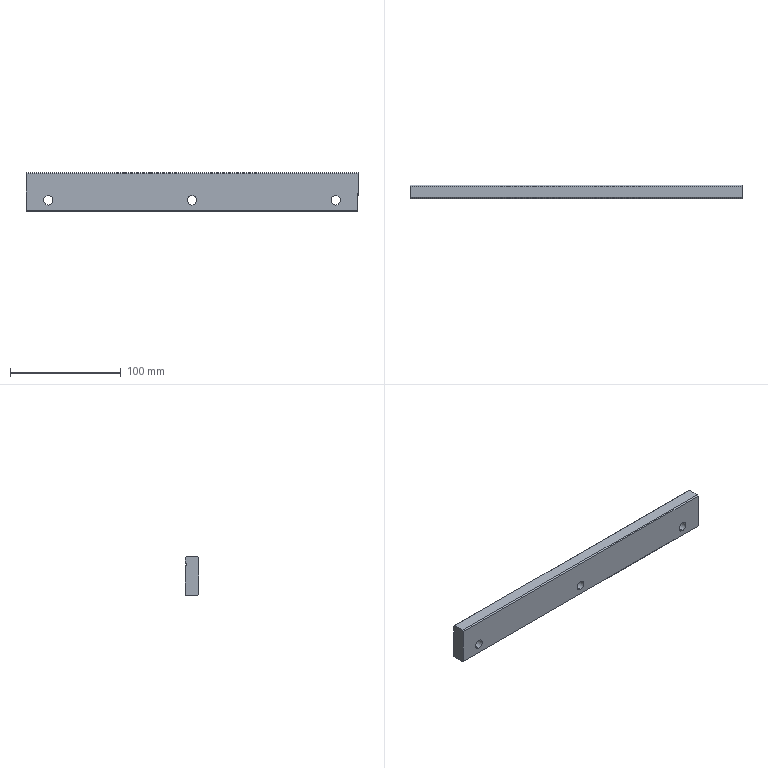Component | SolidWorks | 9LeftPressurePlate-1 | 1 solid | 19 faces | box 300 x 12 x 35 mm | volume 122907 mm3 | plane 13 | cylinder 6 | commonest cylinder face diameters 8.5 x6
build123d program:
from build123d import *

# Parameters (mm, degrees)
SKETCH1_W               = 300
SKETCH1_H               = 35
BOSS_EXTRUDE1_DEPTH     = 12
CUT_EXTRUDE1_DEPTH      = 301.749
CUT_EXTRUDE1_DEPTH_BACK = 301.749
SKETCH2_W               = 2
SKETCH2_H               = 2
CUT_EXTRUDE2_DEPTH      = 152.493
CUT_EXTRUDE2_DEPTH_BACK = 152.493
SKETCH3_R               = 4.25
CHAMFER1_SIZE           = 1


with BuildPart() as part:
    # Sketch1 → Boss-Extrude1 (new body)
    with BuildSketch(Plane(origin=(0, 0, 0), x_dir=(1, 0, 0), z_dir=(0, 1, 0))):
        Rectangle(SKETCH1_W, SKETCH1_H)
    extrude(amount=BOSS_EXTRUDE1_DEPTH)

    # Sketch2 → Cut-Extrude1 (cut, two sides: drawn at the far end of the back side and taken through both)
    with BuildSketch(Plane.ZY.offset(150).offset(-CUT_EXTRUDE1_DEPTH_BACK)):
        with Locations((10.5, 12)):
            Rectangle(SKETCH2_W, SKETCH2_H)
    extrude(amount=CUT_EXTRUDE1_DEPTH + CUT_EXTRUDE1_DEPTH_BACK, mode=Mode.SUBTRACT)

    # Sketch3 → Cut-Extrude2 (cut, two sides: drawn at the far end of the back side and taken through both)
    with BuildSketch(Plane(origin=(0, 12, 0), x_dir=(1, 0, 0), z_dir=(0, 1, 0)).offset(-CUT_EXTRUDE2_DEPTH_BACK)):
        with Locations(Location((-130, 7.5, 0), (0, 0, 270))):
            Circle(SKETCH3_R)
        with Locations(Location((0, 7.5, 0), (0, 0, 270))):
            Circle(SKETCH3_R)
        with Locations(Location((130, 7.5, 0), (0, 0, 270))):
            Circle(SKETCH3_R)
    extrude(amount=CUT_EXTRUDE2_DEPTH + CUT_EXTRUDE2_DEPTH_BACK, mode=Mode.SUBTRACT)

    # Chamfer1
    chamfer1_edges = [part.edges().sort_by_distance(p)[0] for p in [
        (0, 12, 17.5),
        (0, 0, 17.5),
        (0, 0, -17.5),
    ]]
    chamfer(chamfer1_edges, length=CHAMFER1_SIZE)


solid = part.part

# Placed as in the assembly
solid = solid.moved(Location((-4.717, 155, -32.5), (0, 0, 0)))
STEP:
#1=COLOUR_RGB('',0.7922,0.8196,0.9333);
#2=FILL_AREA_STYLE_COLOUR('',#1);
#3=FILL_AREA_STYLE('',(#2));
#4=SURFACE_STYLE_FILL_AREA(#3);
#5=SURFACE_SIDE_STYLE('',(#4));
#6=SURFACE_STYLE_USAGE(.BOTH.,#5);
#7=PRESENTATION_STYLE_ASSIGNMENT((#6));
#8=CARTESIAN_POINT('',(-5.304,6.102,-1.742));
#9=VERTEX_POINT('',#8);
#10=CARTESIAN_POINT('',(-5.304,6.102,-1.407));
#11=VERTEX_POINT('',#10);
#12=CARTESIAN_POINT('',(-5.304,6.102,-1.575));
#13=DIRECTION('',(0.,1.,0.));
#14=DIRECTION('',(0.,0.,1.));
#15=AXIS2_PLACEMENT_3D('',#12,#13,#14);
#16=CIRCLE('',#15,0.1673);
#17=EDGE_CURVE('',#9,#11,#16,.T.);
#18=ORIENTED_EDGE('',*,*,#17,.F.);
#19=CARTESIAN_POINT('',(-5.304,6.575,-1.742));
#20=VERTEX_POINT('',#19);
#21=CARTESIAN_POINT('',(-5.304,6.102,-1.742));
#22=DIRECTION('',(0.,1.,0.));
#23=VECTOR('',#22,39.37);
#24=LINE('',#21,#23);
#25=EDGE_CURVE('',#9,#20,#24,.T.);
#26=ORIENTED_EDGE('',*,*,#25,.T.);
#27=CARTESIAN_POINT('',(-5.304,6.575,-1.407));
#28=VERTEX_POINT('',#27);
#29=CARTESIAN_POINT('',(-5.304,6.575,-1.575));
#30=DIRECTION('',(0.,1.,0.));
#31=DIRECTION('',(0.,0.,1.));
#32=AXIS2_PLACEMENT_3D('',#29,#30,#31);
#33=CIRCLE('',#32,0.1673);
#34=EDGE_CURVE('',#20,#28,#33,.T.);
#35=ORIENTED_EDGE('',*,*,#34,.T.);
#36=CARTESIAN_POINT('',(-5.304,6.102,-1.407));
#37=DIRECTION('',(0.,1.,0.));
#38=VECTOR('',#37,39.37);
#39=LINE('',#36,#38);
#40=EDGE_CURVE('',#11,#28,#39,.T.);
#41=ORIENTED_EDGE('',*,*,#40,.F.);
#42=EDGE_LOOP('',(#18,#26,#35,#41));
#43=FACE_OUTER_BOUND('',#42,.T.);
#44=CARTESIAN_POINT('',(-5.304,6.102,-1.575));
#45=DIRECTION('',(0.,1.,0.));
#46=DIRECTION('',(0.,0.,1.));
#47=AXIS2_PLACEMENT_3D('',#44,#45,#46);
#48=CYLINDRICAL_SURFACE('',#47,0.1673);
#49=ADVANCED_FACE('',(#43),#48,.F.);
#50=CARTESIAN_POINT('',(-0.1857,6.102,-1.742));
#51=VERTEX_POINT('',#50);
#52=CARTESIAN_POINT('',(-0.1857,6.102,-1.407));
#53=VERTEX_POINT('',#52);
#54=CARTESIAN_POINT('',(-0.1857,6.102,-1.575));
#55=DIRECTION('',(0.,1.,0.));
#56=DIRECTION('',(0.,0.,1.));
#57=AXIS2_PLACEMENT_3D('',#54,#55,#56);
#58=CIRCLE('',#57,0.1673);
#59=EDGE_CURVE('',#51,#53,#58,.T.);
#60=ORIENTED_EDGE('',*,*,#59,.F.);
#61=CARTESIAN_POINT('',(-0.1857,6.575,-1.742));
#62=VERTEX_POINT('',#61);
#63=CARTESIAN_POINT('',(-0.1857,6.102,-1.742));
#64=DIRECTION('',(0.,1.,0.));
#65=VECTOR('',#64,39.37);
#66=LINE('',#63,#65);
#67=EDGE_CURVE('',#51,#62,#66,.T.);
#68=ORIENTED_EDGE('',*,*,#67,.T.);
#69=CARTESIAN_POINT('',(-0.1857,6.575,-1.407));
#70=VERTEX_POINT('',#69);
#71=CARTESIAN_POINT('',(-0.1857,6.575,-1.575));
#72=DIRECTION('',(0.,1.,0.));
#73=DIRECTION('',(0.,0.,1.));
#74=AXIS2_PLACEMENT_3D('',#71,#72,#73);
#75=CIRCLE('',#74,0.1673);
#76=EDGE_CURVE('',#62,#70,#75,.T.);
#77=ORIENTED_EDGE('',*,*,#76,.T.);
#78=CARTESIAN_POINT('',(-0.1857,6.102,-1.407));
#79=DIRECTION('',(0.,1.,0.));
#80=VECTOR('',#79,39.37);
#81=LINE('',#78,#80);
#82=EDGE_CURVE('',#53,#70,#81,.T.);
#83=ORIENTED_EDGE('',*,*,#82,.F.);
#84=EDGE_LOOP('',(#60,#68,#77,#83));
#85=FACE_OUTER_BOUND('',#84,.T.);
#86=CARTESIAN_POINT('',(-0.1857,6.102,-1.575));
#87=DIRECTION('',(0.,1.,0.));
#88=DIRECTION('',(0.,0.,1.));
#89=AXIS2_PLACEMENT_3D('',#86,#87,#88);
#90=CYLINDRICAL_SURFACE('',#89,0.1673);
#91=ADVANCED_FACE('',(#85),#90,.F.);
#92=CARTESIAN_POINT('',(4.932,6.102,-1.742));
#93=VERTEX_POINT('',#92);
#94=CARTESIAN_POINT('',(4.932,6.102,-1.407));
#95=VERTEX_POINT('',#94);
#96=CARTESIAN_POINT('',(4.932,6.102,-1.575));
#97=DIRECTION('',(0.,1.,0.));
#98=DIRECTION('',(0.,0.,1.));
#99=AXIS2_PLACEMENT_3D('',#96,#97,#98);
#100=CIRCLE('',#99,0.1673);
#101=EDGE_CURVE('',#93,#95,#100,.T.);
#102=ORIENTED_EDGE('',*,*,#101,.F.);
#103=CARTESIAN_POINT('',(4.932,6.575,-1.742));
#104=VERTEX_POINT('',#103);
#105=CARTESIAN_POINT('',(4.932,6.102,-1.742));
#106=DIRECTION('',(0.,1.,0.));
#107=VECTOR('',#106,39.37);
#108=LINE('',#105,#107);
#109=EDGE_CURVE('',#93,#104,#108,.T.);
#110=ORIENTED_EDGE('',*,*,#109,.T.);
#111=CARTESIAN_POINT('',(4.932,6.575,-1.407));
#112=VERTEX_POINT('',#111);
#113=CARTESIAN_POINT('',(4.932,6.575,-1.575));
#114=DIRECTION('',(0.,1.,0.));
#115=DIRECTION('',(0.,0.,1.));
#116=AXIS2_PLACEMENT_3D('',#113,#114,#115);
#117=CIRCLE('',#116,0.1673);
#118=EDGE_CURVE('',#104,#112,#117,.T.);
#119=ORIENTED_EDGE('',*,*,#118,.T.);
#120=CARTESIAN_POINT('',(4.932,6.102,-1.407));
#121=DIRECTION('',(0.,1.,0.));
#122=VECTOR('',#121,39.37);
#123=LINE('',#120,#122);
#124=EDGE_CURVE('',#95,#112,#123,.T.);
#125=ORIENTED_EDGE('',*,*,#124,.F.);
#126=EDGE_LOOP('',(#102,#110,#119,#125));
#127=FACE_OUTER_BOUND('',#126,.T.);
#128=CARTESIAN_POINT('',(4.932,6.102,-1.575));
#129=DIRECTION('',(0.,1.,0.));
#130=DIRECTION('',(0.,0.,1.));
#131=AXIS2_PLACEMENT_3D('',#128,#129,#130);
#132=CYLINDRICAL_SURFACE('',#131,0.1673);
#133=ADVANCED_FACE('',(#127),#132,.F.);
#134=CARTESIAN_POINT('',(-6.091,6.575,-0.8268));
#135=VERTEX_POINT('',#134);
#136=CARTESIAN_POINT('',(-6.091,6.575,-0.6299));
#137=VERTEX_POINT('',#136);
#138=CARTESIAN_POINT('',(-6.091,6.575,-1.969));
#139=DIRECTION('',(0.,0.,1.));
#140=VECTOR('',#139,39.37);
#141=LINE('',#138,#140);
#142=EDGE_CURVE('',#135,#137,#141,.T.);
#143=ORIENTED_EDGE('',*,*,#142,.T.);
#144=CARTESIAN_POINT('',(5.72,6.575,-0.6299));
#145=VERTEX_POINT('',#144);
#146=CARTESIAN_POINT('',(5.72,6.575,-0.6299));
#147=DIRECTION('',(1.,0.,0.));
#148=VECTOR('',#147,39.37);
#149=LINE('',#146,#148);
#150=EDGE_CURVE('',#137,#145,#149,.T.);
#151=ORIENTED_EDGE('',*,*,#150,.T.);
#152=CARTESIAN_POINT('',(5.72,6.575,-0.8268));
#153=VERTEX_POINT('',#152);
#154=CARTESIAN_POINT('',(5.72,6.575,-1.969));
#155=DIRECTION('',(-0.,0.,-1.));
#156=VECTOR('',#155,39.37);
#157=LINE('',#154,#156);
#158=EDGE_CURVE('',#145,#153,#157,.T.);
#159=ORIENTED_EDGE('',*,*,#158,.T.);
#160=CARTESIAN_POINT('',(-0.1857,6.575,-0.8268));
#161=DIRECTION('',(1.,0.,-0.));
#162=VECTOR('',#161,39.37);
#163=LINE('',#160,#162);
#164=EDGE_CURVE('',#135,#153,#163,.T.);
#165=ORIENTED_EDGE('',*,*,#164,.F.);
#166=EDGE_LOOP('',(#143,#151,#159,#165));
#167=FACE_OUTER_BOUND('',#166,.T.);
#168=CARTESIAN_POINT('',(-0.1857,6.575,-1.28));
#169=DIRECTION('',(0.,1.,0.));
#170=DIRECTION('',(0.,0.,1.));
#171=AXIS2_PLACEMENT_3D('',#168,#169,#170);
#172=PLANE('',#171);
#173=ADVANCED_FACE('',(#167),#172,.T.);
#174=ORIENTED_EDGE('',*,*,#158,.F.);
#175=CARTESIAN_POINT('',(5.72,6.535,-0.5906));
#176=VERTEX_POINT('',#175);
#177=CARTESIAN_POINT('',(5.72,6.575,-0.6299));
#178=DIRECTION('',(0.,-0.7071,0.7071));
#179=VECTOR('',#178,39.37);
#180=LINE('',#177,#179);
#181=EDGE_CURVE('',#145,#176,#180,.T.);
#182=ORIENTED_EDGE('',*,*,#181,.T.);
#183=CARTESIAN_POINT('',(5.72,6.142,-0.5906));
#184=VERTEX_POINT('',#183);
#185=CARTESIAN_POINT('',(5.72,6.575,-0.5906));
#186=DIRECTION('',(0.,-1.,0.));
#187=VECTOR('',#186,39.37);
#188=LINE('',#185,#187);
#189=EDGE_CURVE('',#176,#184,#188,.T.);
#190=ORIENTED_EDGE('',*,*,#189,.T.);
#191=CARTESIAN_POINT('',(5.72,6.102,-0.6299));
#192=VERTEX_POINT('',#191);
#193=CARTESIAN_POINT('',(5.72,6.142,-0.5906));
#194=DIRECTION('',(-0.,-0.7071,-0.7071));
#195=VECTOR('',#194,39.37);
#196=LINE('',#193,#195);
#197=EDGE_CURVE('',#184,#192,#196,.T.);
#198=ORIENTED_EDGE('',*,*,#197,.T.);
#199=CARTESIAN_POINT('',(5.72,6.102,-1.929));
#200=VERTEX_POINT('',#199);
#201=CARTESIAN_POINT('',(5.72,6.102,-1.969));
#202=DIRECTION('',(-0.,0.,-1.));
#203=VECTOR('',#202,39.37);
#204=LINE('',#201,#203);
#205=EDGE_CURVE('',#192,#200,#204,.T.);
#206=ORIENTED_EDGE('',*,*,#205,.T.);
#207=CARTESIAN_POINT('',(5.72,6.142,-1.969));
#208=VERTEX_POINT('',#207);
#209=CARTESIAN_POINT('',(5.72,6.142,-1.969));
#210=DIRECTION('',(-0.,0.7071,-0.7071));
#211=VECTOR('',#210,39.37);
#212=LINE('',#209,#211);
#213=EDGE_CURVE('',#200,#208,#212,.T.);
#214=ORIENTED_EDGE('',*,*,#213,.T.);
#215=CARTESIAN_POINT('',(5.72,6.575,-1.969));
#216=VERTEX_POINT('',#215);
#217=CARTESIAN_POINT('',(5.72,6.575,-1.969));
#218=DIRECTION('',(0.,-1.,0.));
#219=VECTOR('',#218,39.37);
#220=LINE('',#217,#219);
#221=EDGE_CURVE('',#216,#208,#220,.T.);
#222=ORIENTED_EDGE('',*,*,#221,.F.);
#223=CARTESIAN_POINT('',(5.72,6.575,-0.9055));
#224=VERTEX_POINT('',#223);
#225=CARTESIAN_POINT('',(5.72,6.575,-1.969));
#226=DIRECTION('',(-0.,0.,-1.));
#227=VECTOR('',#226,39.37);
#228=LINE('',#225,#227);
#229=EDGE_CURVE('',#224,#216,#228,.T.);
#230=ORIENTED_EDGE('',*,*,#229,.F.);
#231=CARTESIAN_POINT('',(5.72,6.535,-0.9055));
#232=VERTEX_POINT('',#231);
#233=CARTESIAN_POINT('',(5.72,6.614,-0.9055));
#234=DIRECTION('',(0.,-1.,0.));
#235=VECTOR('',#234,39.37);
#236=LINE('',#233,#235);
#237=EDGE_CURVE('',#224,#232,#236,.T.);
#238=ORIENTED_EDGE('',*,*,#237,.T.);
#239=CARTESIAN_POINT('',(5.72,6.535,-0.8268));
#240=VERTEX_POINT('',#239);
#241=CARTESIAN_POINT('',(5.72,6.535,-0.9055));
#242=DIRECTION('',(0.,0.,1.));
#243=VECTOR('',#242,39.37);
#244=LINE('',#241,#243);
#245=EDGE_CURVE('',#232,#240,#244,.T.);
#246=ORIENTED_EDGE('',*,*,#245,.T.);
#247=CARTESIAN_POINT('',(5.72,6.614,-0.8268));
#248=DIRECTION('',(0.,1.,0.));
#249=VECTOR('',#248,39.37);
#250=LINE('',#247,#249);
#251=EDGE_CURVE('',#240,#153,#250,.T.);
#252=ORIENTED_EDGE('',*,*,#251,.T.);
#253=EDGE_LOOP('',(#174,#182,#190,#198,#206,#214,#222,#230,#238,#246,#252));
#254=FACE_OUTER_BOUND('',#253,.T.);
#255=CARTESIAN_POINT('',(5.72,6.575,-1.969));
#256=DIRECTION('',(-1.,0.,0.));
#257=DIRECTION('',(0.,0.,1.));
#258=AXIS2_PLACEMENT_3D('',#255,#256,#257);
#259=PLANE('',#258);
#260=ADVANCED_FACE('',(#254),#259,.F.);
#261=ORIENTED_EDGE('',*,*,#221,.T.);
#262=CARTESIAN_POINT('',(-6.091,6.142,-1.969));
#263=VERTEX_POINT('',#262);
#264=CARTESIAN_POINT('',(-6.091,6.142,-1.969));
#265=DIRECTION('',(-1.,0.,0.));
#266=VECTOR('',#265,39.37);
#267=LINE('',#264,#266);
#268=EDGE_CURVE('',#208,#263,#267,.T.);
#269=ORIENTED_EDGE('',*,*,#268,.T.);
#270=CARTESIAN_POINT('',(-6.091,6.575,-1.969));
#271=VERTEX_POINT('',#270);
#272=CARTESIAN_POINT('',(-6.091,6.575,-1.969));
#273=DIRECTION('',(0.,-1.,0.));
#274=VECTOR('',#273,39.37);
#275=LINE('',#272,#274);
#276=EDGE_CURVE('',#271,#263,#275,.T.);
#277=ORIENTED_EDGE('',*,*,#276,.F.);
#278=CARTESIAN_POINT('',(-6.091,6.575,-1.969));
#279=DIRECTION('',(-1.,0.,0.));
#280=VECTOR('',#279,39.37);
#281=LINE('',#278,#280);
#282=EDGE_CURVE('',#216,#271,#281,.T.);
#283=ORIENTED_EDGE('',*,*,#282,.F.);
#284=EDGE_LOOP('',(#261,#269,#277,#283));
#285=FACE_OUTER_BOUND('',#284,.T.);
#286=CARTESIAN_POINT('',(-6.091,6.575,-1.969));
#287=DIRECTION('',(0.,0.,1.));
#288=DIRECTION('',(1.,0.,0.));
#289=AXIS2_PLACEMENT_3D('',#286,#287,#288);
#290=PLANE('',#289);
#291=ADVANCED_FACE('',(#285),#290,.F.);
#292=CARTESIAN_POINT('',(-6.091,6.535,-0.5906));
#293=VERTEX_POINT('',#292);
#294=CARTESIAN_POINT('',(-6.091,6.142,-0.5906));
#295=VERTEX_POINT('',#294);
#296=CARTESIAN_POINT('',(-6.091,6.575,-0.5906));
#297=DIRECTION('',(0.,-1.,0.));
#298=VECTOR('',#297,39.37);
#299=LINE('',#296,#298);
#300=EDGE_CURVE('',#293,#295,#299,.T.);
#301=ORIENTED_EDGE('',*,*,#300,.F.);
#302=CARTESIAN_POINT('',(-6.091,6.575,-0.6299));
#303=DIRECTION('',(-0.,0.7071,-0.7071));
#304=VECTOR('',#303,39.37);
#305=LINE('',#302,#304);
#306=EDGE_CURVE('',#293,#137,#305,.T.);
#307=ORIENTED_EDGE('',*,*,#306,.T.);
#308=ORIENTED_EDGE('',*,*,#142,.F.);
#309=CARTESIAN_POINT('',(-6.091,6.535,-0.8268));
#310=VERTEX_POINT('',#309);
#311=CARTESIAN_POINT('',(-6.091,6.575,-0.8268));
#312=DIRECTION('',(0.,-1.,0.));
#313=VECTOR('',#312,39.37);
#314=LINE('',#311,#313);
#315=EDGE_CURVE('',#135,#310,#314,.T.);
#316=ORIENTED_EDGE('',*,*,#315,.T.);
#317=CARTESIAN_POINT('',(-6.091,6.535,-0.9055));
#318=VERTEX_POINT('',#317);
#319=CARTESIAN_POINT('',(-6.091,6.535,-1.969));
#320=DIRECTION('',(-0.,0.,-1.));
#321=VECTOR('',#320,39.37);
#322=LINE('',#319,#321);
#323=EDGE_CURVE('',#310,#318,#322,.T.);
#324=ORIENTED_EDGE('',*,*,#323,.T.);
#325=CARTESIAN_POINT('',(-6.091,6.575,-0.9055));
#326=VERTEX_POINT('',#325);
#327=CARTESIAN_POINT('',(-6.091,6.575,-0.9055));
#328=DIRECTION('',(0.,1.,0.));
#329=VECTOR('',#328,39.37);
#330=LINE('',#327,#329);
#331=EDGE_CURVE('',#318,#326,#330,.T.);
#332=ORIENTED_EDGE('',*,*,#331,.T.);
#333=CARTESIAN_POINT('',(-6.091,6.575,-1.969));
#334=DIRECTION('',(0.,0.,1.));
#335=VECTOR('',#334,39.37);
#336=LINE('',#333,#335);
#337=EDGE_CURVE('',#271,#326,#336,.T.);
#338=ORIENTED_EDGE('',*,*,#337,.F.);
#339=ORIENTED_EDGE('',*,*,#276,.T.);
#340=CARTESIAN_POINT('',(-6.091,6.102,-1.929));
#341=VERTEX_POINT('',#340);
#342=CARTESIAN_POINT('',(-6.091,6.142,-1.969));
#343=DIRECTION('',(0.,-0.7071,0.7071));
#344=VECTOR('',#343,39.37);
#345=LINE('',#342,#344);
#346=EDGE_CURVE('',#263,#341,#345,.T.);
#347=ORIENTED_EDGE('',*,*,#346,.T.);
#348=CARTESIAN_POINT('',(-6.091,6.102,-0.6299));
#349=VERTEX_POINT('',#348);
#350=CARTESIAN_POINT('',(-6.091,6.102,-1.969));
#351=DIRECTION('',(0.,0.,1.));
#352=VECTOR('',#351,39.37);
#353=LINE('',#350,#352);
#354=EDGE_CURVE('',#341,#349,#353,.T.);
#355=ORIENTED_EDGE('',*,*,#354,.T.);
#356=CARTESIAN_POINT('',(-6.091,6.142,-0.5906));
#357=DIRECTION('',(0.,0.7071,0.7071));
#358=VECTOR('',#357,39.37);
#359=LINE('',#356,#358);
#360=EDGE_CURVE('',#349,#295,#359,.T.);
#361=ORIENTED_EDGE('',*,*,#360,.T.);
#362=EDGE_LOOP('',(#301,#307,#308,#316,#324,#332,#338,#339,#347,#355,#361));
#363=FACE_OUTER_BOUND('',#362,.T.);
#364=CARTESIAN_POINT('',(-6.091,6.575,-1.969));
#365=DIRECTION('',(1.,0.,-0.));
#366=DIRECTION('',(-0.,0.,-1.));
#367=AXIS2_PLACEMENT_3D('',#364,#365,#366);
#368=PLANE('',#367);
#369=ADVANCED_FACE('',(#363),#368,.F.);
#370=ORIENTED_EDGE('',*,*,#189,.F.);
#371=CARTESIAN_POINT('',(-6.091,6.535,-0.5906));
#372=DIRECTION('',(-1.,0.,0.));
#373=VECTOR('',#372,39.37);
#374=LINE('',#371,#373);
#375=EDGE_CURVE('',#176,#293,#374,.T.);
#376=ORIENTED_EDGE('',*,*,#375,.T.);
#377=ORIENTED_EDGE('',*,*,#300,.T.);
#378=CARTESIAN_POINT('',(-6.091,6.142,-0.5906));
#379=DIRECTION('',(1.,0.,0.));
#380=VECTOR('',#379,39.37);
#381=LINE('',#378,#380);
#382=EDGE_CURVE('',#295,#184,#381,.T.);
#383=ORIENTED_EDGE('',*,*,#382,.T.);
#384=EDGE_LOOP('',(#370,#376,#377,#383));
#385=FACE_OUTER_BOUND('',#384,.T.);
#386=CARTESIAN_POINT('',(-6.091,6.575,-0.5906));
#387=DIRECTION('',(0.,0.,-1.));
#388=DIRECTION('',(-1.,0.,0.));
#389=AXIS2_PLACEMENT_3D('',#386,#387,#388);
#390=PLANE('',#389);
#391=ADVANCED_FACE('',(#385),#390,.F.);
#392=CARTESIAN_POINT('',(-5.304,6.575,-1.575));
#393=DIRECTION('',(0.,1.,0.));
#394=DIRECTION('',(0.,0.,1.));
#395=AXIS2_PLACEMENT_3D('',#392,#393,#394);
#396=CIRCLE('',#395,0.1673);
#397=EDGE_CURVE('',#28,#20,#396,.T.);
#398=ORIENTED_EDGE('',*,*,#397,.F.);
#399=ORIENTED_EDGE('',*,*,#34,.F.);
#400=EDGE_LOOP('',(#398,#399));
#401=FACE_BOUND('',#400,.T.);
#402=CARTESIAN_POINT('',(-0.1857,6.575,-1.575));
#403=DIRECTION('',(0.,1.,0.));
#404=DIRECTION('',(0.,0.,1.));
#405=AXIS2_PLACEMENT_3D('',#402,#403,#404);
#406=CIRCLE('',#405,0.1673);
#407=EDGE_CURVE('',#70,#62,#406,.T.);
#408=ORIENTED_EDGE('',*,*,#407,.F.);
#409=ORIENTED_EDGE('',*,*,#76,.F.);
#410=EDGE_LOOP('',(#408,#409));
#411=FACE_BOUND('',#410,.T.);
#412=CARTESIAN_POINT('',(4.932,6.575,-1.575));
#413=DIRECTION('',(0.,1.,0.));
#414=DIRECTION('',(0.,0.,1.));
#415=AXIS2_PLACEMENT_3D('',#412,#413,#414);
#416=CIRCLE('',#415,0.1673);
#417=EDGE_CURVE('',#112,#104,#416,.T.);
#418=ORIENTED_EDGE('',*,*,#417,.F.);
#419=ORIENTED_EDGE('',*,*,#118,.F.);
#420=EDGE_LOOP('',(#418,#419));
#421=FACE_BOUND('',#420,.T.);
#422=CARTESIAN_POINT('',(-0.1857,6.575,-0.9055));
#423=DIRECTION('',(-1.,0.,0.));
#424=VECTOR('',#423,39.37);
#425=LINE('',#422,#424);
#426=EDGE_CURVE('',#224,#326,#425,.T.);
#427=ORIENTED_EDGE('',*,*,#426,.F.);
#428=ORIENTED_EDGE('',*,*,#229,.T.);
#429=ORIENTED_EDGE('',*,*,#282,.T.);
#430=ORIENTED_EDGE('',*,*,#337,.T.);
#431=EDGE_LOOP('',(#427,#428,#429,#430));
#432=FACE_OUTER_BOUND('',#431,.T.);
#433=CARTESIAN_POINT('',(-0.1857,6.575,-1.28));
#434=DIRECTION('',(0.,1.,0.));
#435=DIRECTION('',(0.,0.,1.));
#436=AXIS2_PLACEMENT_3D('',#433,#434,#435);
#437=PLANE('',#436);
#438=ADVANCED_FACE('',(#401,#411,#421,#432),#437,.T.);
#439=CARTESIAN_POINT('',(-5.304,6.102,-1.575));
#440=DIRECTION('',(0.,1.,0.));
#441=DIRECTION('',(0.,0.,1.));
#442=AXIS2_PLACEMENT_3D('',#439,#440,#441);
#443=CIRCLE('',#442,0.1673);
#444=EDGE_CURVE('',#11,#9,#443,.T.);
#445=ORIENTED_EDGE('',*,*,#444,.T.);
#446=ORIENTED_EDGE('',*,*,#17,.T.);
#447=EDGE_LOOP('',(#445,#446));
#448=FACE_BOUND('',#447,.T.);
#449=CARTESIAN_POINT('',(-0.1857,6.102,-1.575));
#450=DIRECTION('',(0.,1.,0.));
#451=DIRECTION('',(0.,0.,1.));
#452=AXIS2_PLACEMENT_3D('',#449,#450,#451);
#453=CIRCLE('',#452,0.1673);
#454=EDGE_CURVE('',#53,#51,#453,.T.);
#455=ORIENTED_EDGE('',*,*,#454,.T.);
#456=ORIENTED_EDGE('',*,*,#59,.T.);
#457=EDGE_LOOP('',(#455,#456));
#458=FACE_BOUND('',#457,.T.);
#459=CARTESIAN_POINT('',(4.932,6.102,-1.575));
#460=DIRECTION('',(0.,1.,0.));
#461=DIRECTION('',(0.,0.,1.));
#462=AXIS2_PLACEMENT_3D('',#459,#460,#461);
#463=CIRCLE('',#462,0.1673);
#464=EDGE_CURVE('',#95,#93,#463,.T.);
#465=ORIENTED_EDGE('',*,*,#464,.T.);
#466=ORIENTED_EDGE('',*,*,#101,.T.);
#467=EDGE_LOOP('',(#465,#466));
#468=FACE_BOUND('',#467,.T.);
#469=ORIENTED_EDGE('',*,*,#205,.F.);
#470=CARTESIAN_POINT('',(-0.1857,6.102,-0.6299));
#471=DIRECTION('',(-1.,0.,0.));
#472=VECTOR('',#471,39.37);
#473=LINE('',#470,#472);
#474=EDGE_CURVE('',#192,#349,#473,.T.);
#475=ORIENTED_EDGE('',*,*,#474,.T.);
#476=ORIENTED_EDGE('',*,*,#354,.F.);
#477=CARTESIAN_POINT('',(-0.1857,6.102,-1.929));
#478=DIRECTION('',(1.,0.,0.));
#479=VECTOR('',#478,39.37);
#480=LINE('',#477,#479);
#481=EDGE_CURVE('',#341,#200,#480,.T.);
#482=ORIENTED_EDGE('',*,*,#481,.T.);
#483=EDGE_LOOP('',(#469,#475,#476,#482));
#484=FACE_OUTER_BOUND('',#483,.T.);
#485=CARTESIAN_POINT('',(-0.1857,6.102,-1.28));
#486=DIRECTION('',(0.,1.,0.));
#487=DIRECTION('',(0.,0.,1.));
#488=AXIS2_PLACEMENT_3D('',#485,#486,#487);
#489=PLANE('',#488);
#490=ADVANCED_FACE('',(#448,#458,#468,#484),#489,.F.);
#491=CARTESIAN_POINT('',(5.72,6.535,-0.8268));
#492=DIRECTION('',(-1.,0.,0.));
#493=VECTOR('',#492,39.37);
#494=LINE('',#491,#493);
#495=EDGE_CURVE('',#240,#310,#494,.T.);
#496=ORIENTED_EDGE('',*,*,#495,.F.);
#497=ORIENTED_EDGE('',*,*,#245,.F.);
#498=CARTESIAN_POINT('',(5.72,6.535,-0.9055));
#499=DIRECTION('',(-1.,0.,0.));
#500=VECTOR('',#499,39.37);
#501=LINE('',#498,#500);
#502=EDGE_CURVE('',#232,#318,#501,.T.);
#503=ORIENTED_EDGE('',*,*,#502,.T.);
#504=ORIENTED_EDGE('',*,*,#323,.F.);
#505=EDGE_LOOP('',(#496,#497,#503,#504));
#506=FACE_OUTER_BOUND('',#505,.T.);
#507=CARTESIAN_POINT('',(5.72,6.535,-0.9055));
#508=DIRECTION('',(0.,-1.,0.));
#509=DIRECTION('',(0.,0.,-1.));
#510=AXIS2_PLACEMENT_3D('',#507,#508,#509);
#511=PLANE('',#510);
#512=ADVANCED_FACE('',(#506),#511,.F.);
#513=ORIENTED_EDGE('',*,*,#164,.T.);
#514=ORIENTED_EDGE('',*,*,#251,.F.);
#515=ORIENTED_EDGE('',*,*,#495,.T.);
#516=ORIENTED_EDGE('',*,*,#315,.F.);
#517=EDGE_LOOP('',(#513,#514,#515,#516));
#518=FACE_OUTER_BOUND('',#517,.T.);
#519=CARTESIAN_POINT('',(5.72,6.614,-0.8268));
#520=DIRECTION('',(0.,0.,1.));
#521=DIRECTION('',(1.,0.,-0.));
#522=AXIS2_PLACEMENT_3D('',#519,#520,#521);
#523=PLANE('',#522);
#524=ADVANCED_FACE('',(#518),#523,.F.);
#525=ORIENTED_EDGE('',*,*,#502,.F.);
#526=ORIENTED_EDGE('',*,*,#237,.F.);
#527=ORIENTED_EDGE('',*,*,#426,.T.);
#528=ORIENTED_EDGE('',*,*,#331,.F.);
#529=EDGE_LOOP('',(#525,#526,#527,#528));
#530=FACE_OUTER_BOUND('',#529,.T.);
#531=CARTESIAN_POINT('',(5.72,6.614,-0.9055));
#532=DIRECTION('',(-0.,0.,-1.));
#533=DIRECTION('',(-1.,0.,0.));
#534=AXIS2_PLACEMENT_3D('',#531,#532,#533);
#535=PLANE('',#534);
#536=ADVANCED_FACE('',(#530),#535,.F.);
#537=ORIENTED_EDGE('',*,*,#109,.F.);
#538=ORIENTED_EDGE('',*,*,#464,.F.);
#539=ORIENTED_EDGE('',*,*,#124,.T.);
#540=ORIENTED_EDGE('',*,*,#417,.T.);
#541=EDGE_LOOP('',(#537,#538,#539,#540));
#542=FACE_OUTER_BOUND('',#541,.T.);
#543=CARTESIAN_POINT('',(4.932,6.102,-1.575));
#544=DIRECTION('',(0.,1.,0.));
#545=DIRECTION('',(0.,0.,1.));
#546=AXIS2_PLACEMENT_3D('',#543,#544,#545);
#547=CYLINDRICAL_SURFACE('',#546,0.1673);
#548=ADVANCED_FACE('',(#542),#547,.F.);
#549=ORIENTED_EDGE('',*,*,#67,.F.);
#550=ORIENTED_EDGE('',*,*,#454,.F.);
#551=ORIENTED_EDGE('',*,*,#82,.T.);
#552=ORIENTED_EDGE('',*,*,#407,.T.);
#553=EDGE_LOOP('',(#549,#550,#551,#552));
#554=FACE_OUTER_BOUND('',#553,.T.);
#555=CARTESIAN_POINT('',(-0.1857,6.102,-1.575));
#556=DIRECTION('',(0.,1.,0.));
#557=DIRECTION('',(0.,0.,1.));
#558=AXIS2_PLACEMENT_3D('',#555,#556,#557);
#559=CYLINDRICAL_SURFACE('',#558,0.1673);
#560=ADVANCED_FACE('',(#554),#559,.F.);
#561=ORIENTED_EDGE('',*,*,#25,.F.);
#562=ORIENTED_EDGE('',*,*,#444,.F.);
#563=ORIENTED_EDGE('',*,*,#40,.T.);
#564=ORIENTED_EDGE('',*,*,#397,.T.);
#565=EDGE_LOOP('',(#561,#562,#563,#564));
#566=FACE_OUTER_BOUND('',#565,.T.);
#567=CARTESIAN_POINT('',(-5.304,6.102,-1.575));
#568=DIRECTION('',(0.,1.,0.));
#569=DIRECTION('',(0.,0.,1.));
#570=AXIS2_PLACEMENT_3D('',#567,#568,#569);
#571=CYLINDRICAL_SURFACE('',#570,0.1673);
#572=ADVANCED_FACE('',(#566),#571,.F.);
#573=ORIENTED_EDGE('',*,*,#306,.F.);
#574=ORIENTED_EDGE('',*,*,#375,.F.);
#575=ORIENTED_EDGE('',*,*,#181,.F.);
#576=ORIENTED_EDGE('',*,*,#150,.F.);
#577=EDGE_LOOP('',(#573,#574,#575,#576));
#578=FACE_OUTER_BOUND('',#577,.T.);
#579=CARTESIAN_POINT('',(-0.1857,6.575,-0.6299));
#580=DIRECTION('',(0.,0.7071,0.7071));
#581=DIRECTION('',(-1.,0.,0.));
#582=AXIS2_PLACEMENT_3D('',#579,#580,#581);
#583=PLANE('',#582);
#584=ADVANCED_FACE('',(#578),#583,.T.);
#585=ORIENTED_EDGE('',*,*,#360,.F.);
#586=ORIENTED_EDGE('',*,*,#474,.F.);
#587=ORIENTED_EDGE('',*,*,#197,.F.);
#588=ORIENTED_EDGE('',*,*,#382,.F.);
#589=EDGE_LOOP('',(#585,#586,#587,#588));
#590=FACE_OUTER_BOUND('',#589,.T.);
#591=CARTESIAN_POINT('',(-6.091,6.142,-0.5906));
#592=DIRECTION('',(0.,0.7071,-0.7071));
#593=DIRECTION('',(1.,0.,0.));
#594=AXIS2_PLACEMENT_3D('',#591,#592,#593);
#595=PLANE('',#594);
#596=ADVANCED_FACE('',(#590),#595,.F.);
#597=ORIENTED_EDGE('',*,*,#213,.F.);
#598=ORIENTED_EDGE('',*,*,#481,.F.);
#599=ORIENTED_EDGE('',*,*,#346,.F.);
#600=ORIENTED_EDGE('',*,*,#268,.F.);
#601=EDGE_LOOP('',(#597,#598,#599,#600));
#602=FACE_OUTER_BOUND('',#601,.T.);
#603=CARTESIAN_POINT('',(-6.091,6.142,-1.969));
#604=DIRECTION('',(0.,0.7071,0.7071));
#605=DIRECTION('',(-1.,0.,0.));
#606=AXIS2_PLACEMENT_3D('',#603,#604,#605);
#607=PLANE('',#606);
#608=ADVANCED_FACE('',(#602),#607,.F.);
#609=CLOSED_SHELL('',(#49,#91,#133,#173,#260,#291,#369,#391,#438,#490,#512,#524,#536,#548,#560,#572,#584,#596,#608));
#610=MANIFOLD_SOLID_BREP('',#609);
#611=STYLED_ITEM('',(#7),#610);
#612=PRESENTATION_LAYER_ASSIGNMENT('','',(#611));
#613=(LENGTH_UNIT()NAMED_UNIT(*)SI_UNIT($,.METRE.));
#614=LENGTH_MEASURE_WITH_UNIT(LENGTH_MEASURE(0.0254),#613);
#615=DIMENSIONAL_EXPONENTS(1.,0.,0.,0.,0.,0.,0.);
#616=(CONVERSION_BASED_UNIT('',#614)LENGTH_UNIT()NAMED_UNIT(#615));
#617=UNCERTAINTY_MEASURE_WITH_UNIT(LENGTH_MEASURE(0.00001),#616,'','');
#618=(NAMED_UNIT(*)PLANE_ANGLE_UNIT()SI_UNIT($,.RADIAN.));
#619=(NAMED_UNIT(*)SI_UNIT($,.STERADIAN.)SOLID_ANGLE_UNIT());
#620=(GEOMETRIC_REPRESENTATION_CONTEXT(3)GLOBAL_UNCERTAINTY_ASSIGNED_CONTEXT((#617))GLOBAL_UNIT_ASSIGNED_CONTEXT((#616,#618,#619))REPRESENTATION_CONTEXT('',''));
#621=MECHANICAL_DESIGN_GEOMETRIC_PRESENTATION_REPRESENTATION('',(#611),#620);
#622=CARTESIAN_POINT('',(0.,0.,0.));
#623=DIRECTION('',(0.,0.,1.));
#624=DIRECTION('',(1.,0.,0.));
#625=AXIS2_PLACEMENT_3D('',#622,#623,#624);
#626=(LENGTH_UNIT()NAMED_UNIT(*)SI_UNIT($,.METRE.));
#627=LENGTH_MEASURE_WITH_UNIT(LENGTH_MEASURE(0.0254),#626);
#628=DIMENSIONAL_EXPONENTS(1.,0.,0.,0.,0.,0.,0.);
#629=(CONVERSION_BASED_UNIT('',#627)LENGTH_UNIT()NAMED_UNIT(#628));
#630=UNCERTAINTY_MEASURE_WITH_UNIT(LENGTH_MEASURE(0.00001),#629,'','');
#631=(NAMED_UNIT(*)PLANE_ANGLE_UNIT()SI_UNIT($,.RADIAN.));
#632=(NAMED_UNIT(*)SI_UNIT($,.STERADIAN.)SOLID_ANGLE_UNIT());
#633=(GEOMETRIC_REPRESENTATION_CONTEXT(3)GLOBAL_UNCERTAINTY_ASSIGNED_CONTEXT((#630))GLOBAL_UNIT_ASSIGNED_CONTEXT((#629,#631,#632))REPRESENTATION_CONTEXT('',''));
#634=ADVANCED_BREP_SHAPE_REPRESENTATION('',(#610,#625),#633);